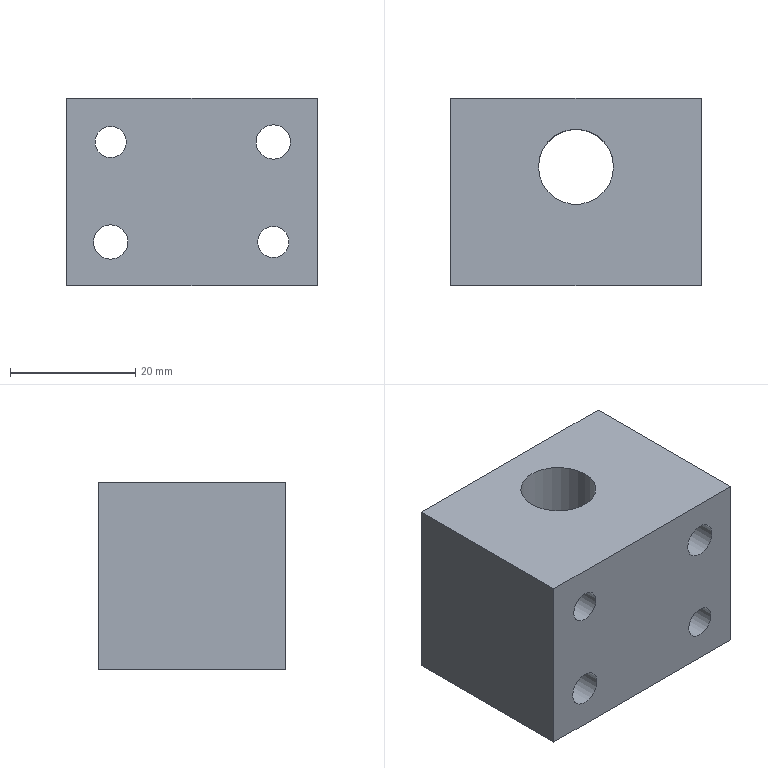Component | NX | ROUND_GUIDE_BLOCK | 1 solid | 19 faces | volume 29231 mm3 | plane 10 | cylinder 9 | commonest cylinder face diameters 5.5 x4 10 x2 5 x2 12 x1